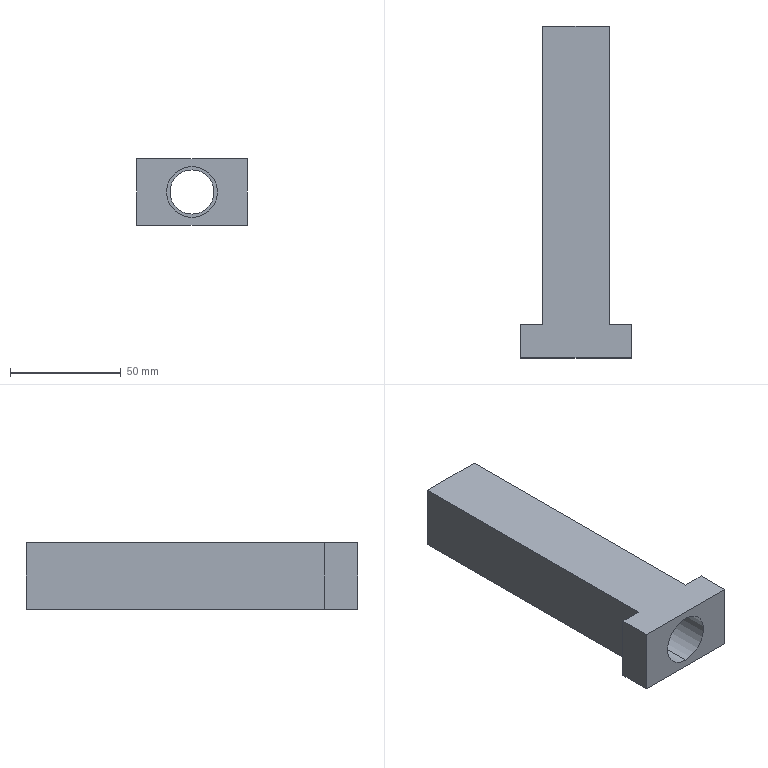Component | SolidWorks | Nut-1 | 1 solid | 15 faces | box 50 x 150 x 30 mm | volume 85731 mm3 | plane 11 | cylinder 4 | commonest cylinder face diameters 20 x2 23 x2
build123d program:
from build123d import *

# Parameters (mm, degrees)
SKETCH1_W           = 50
SKETCH1_H           = 30
BOSS_EXTRUDE1_DEPTH = 15
SKETCH2_W           = 30
SKETCH2_H           = 30
BOSS_EXTRUDE2_DEPTH = 135
CUT_EXTRUDE1_START  = -40
SKETCH3_R           = 11.5
CUT_EXTRUDE1_DEPTH  = 113.807
M20_TAPPED_HOLE1_D  = 20


with BuildPart() as part:
    # Sketch1 → Boss-Extrude1 (new body)
    with BuildSketch(Plane(origin=(0, 0, 0), x_dir=(1, 0, 0), z_dir=(0, 1, 0))):
        Rectangle(SKETCH1_W, SKETCH1_H)
    extrude(amount=BOSS_EXTRUDE1_DEPTH)

    # Sketch2 → Boss-Extrude2 (add)
    with BuildSketch(Plane(origin=(0, 15, 0), x_dir=(1, 0, 0), z_dir=(0, 1, 0))):
        Rectangle(SKETCH2_W, SKETCH2_H)
    extrude(amount=BOSS_EXTRUDE2_DEPTH)

    # Sketch3 → Cut-Extrude1 (cut, through all)
    with BuildSketch(Plane(origin=(0, 150, 0), x_dir=(1, 0, 0), z_dir=(0, 1, 0)).offset(CUT_EXTRUDE1_START)):
        with Locations(Location((0, 0, 0), (0, 0, 270))):
            Circle(SKETCH3_R)
    extrude(amount=-CUT_EXTRUDE1_DEPTH, mode=Mode.SUBTRACT)

    # M20 Tapped Hole1 (through all)
    with Locations(Plane(origin=(0, 150, 0), x_dir=(1, 0, 0), z_dir=(0, 1, 0))):
        with Locations((0, 0)):
            Hole(M20_TAPPED_HOLE1_D / 2)


solid = part.part

# Placed as in the assembly
solid = solid.moved(Location((-29.507, -119.411, 458), (0, 0, 0)))
STEP:
#1=COLOUR_RGB('',0.7922,0.8196,0.9333);
#2=FILL_AREA_STYLE_COLOUR('',#1);
#3=FILL_AREA_STYLE('',(#2));
#4=SURFACE_STYLE_FILL_AREA(#3);
#5=SURFACE_SIDE_STYLE('',(#4));
#6=SURFACE_STYLE_USAGE(.BOTH.,#5);
#7=PRESENTATION_STYLE_ASSIGNMENT((#6));
#8=CARTESIAN_POINT('',(-1.162,-0.3705,17.638));
#9=VERTEX_POINT('',#8);
#10=CARTESIAN_POINT('',(-1.162,-0.3705,18.425));
#11=VERTEX_POINT('',#10);
#12=CARTESIAN_POINT('',(-1.162,-0.3705,18.031));
#13=DIRECTION('',(0.,1.,0.));
#14=DIRECTION('',(0.,0.,1.));
#15=AXIS2_PLACEMENT_3D('',#12,#13,#14);
#16=CIRCLE('',#15,0.3937);
#17=EDGE_CURVE('',#9,#11,#16,.T.);
#18=ORIENTED_EDGE('',*,*,#17,.F.);
#19=CARTESIAN_POINT('',(-1.162,1.204,17.638));
#20=VERTEX_POINT('',#19);
#21=CARTESIAN_POINT('',(-1.162,1.204,17.638));
#22=DIRECTION('',(0.,1.,0.));
#23=VECTOR('',#22,39.37);
#24=LINE('',#21,#23);
#25=EDGE_CURVE('',#9,#20,#24,.T.);
#26=ORIENTED_EDGE('',*,*,#25,.T.);
#27=CARTESIAN_POINT('',(-1.162,1.204,18.425));
#28=VERTEX_POINT('',#27);
#29=CARTESIAN_POINT('',(-1.162,1.204,18.031));
#30=DIRECTION('',(0.,1.,0.));
#31=DIRECTION('',(0.,0.,1.));
#32=AXIS2_PLACEMENT_3D('',#29,#30,#31);
#33=CIRCLE('',#32,0.3937);
#34=EDGE_CURVE('',#20,#28,#33,.T.);
#35=ORIENTED_EDGE('',*,*,#34,.T.);
#36=CARTESIAN_POINT('',(-1.162,1.204,18.425));
#37=DIRECTION('',(0.,1.,0.));
#38=VECTOR('',#37,39.37);
#39=LINE('',#36,#38);
#40=EDGE_CURVE('',#11,#28,#39,.T.);
#41=ORIENTED_EDGE('',*,*,#40,.F.);
#42=EDGE_LOOP('',(#18,#26,#35,#41));
#43=FACE_OUTER_BOUND('',#42,.T.);
#44=CARTESIAN_POINT('',(-1.162,1.204,18.031));
#45=DIRECTION('',(0.,1.,0.));
#46=DIRECTION('',(0.,0.,1.));
#47=AXIS2_PLACEMENT_3D('',#44,#45,#46);
#48=CYLINDRICAL_SURFACE('',#47,0.3937);
#49=ADVANCED_FACE('',(#43),#48,.F.);
#50=CARTESIAN_POINT('',(-1.162,-4.701,17.579));
#51=VERTEX_POINT('',#50);
#52=CARTESIAN_POINT('',(-1.162,-4.701,18.484));
#53=VERTEX_POINT('',#52);
#54=CARTESIAN_POINT('',(-1.162,-4.701,18.031));
#55=DIRECTION('',(0.,1.,0.));
#56=DIRECTION('',(0.,0.,1.));
#57=AXIS2_PLACEMENT_3D('',#54,#55,#56);
#58=CIRCLE('',#57,0.4528);
#59=EDGE_CURVE('',#51,#53,#58,.T.);
#60=ORIENTED_EDGE('',*,*,#59,.F.);
#61=CARTESIAN_POINT('',(-1.162,-0.3705,17.579));
#62=VERTEX_POINT('',#61);
#63=CARTESIAN_POINT('',(-1.162,-4.701,17.579));
#64=DIRECTION('',(0.,1.,0.));
#65=VECTOR('',#64,39.37);
#66=LINE('',#63,#65);
#67=EDGE_CURVE('',#51,#62,#66,.T.);
#68=ORIENTED_EDGE('',*,*,#67,.T.);
#69=CARTESIAN_POINT('',(-1.162,-0.3705,18.484));
#70=VERTEX_POINT('',#69);
#71=CARTESIAN_POINT('',(-1.162,-0.3705,18.031));
#72=DIRECTION('',(0.,1.,0.));
#73=DIRECTION('',(0.,0.,1.));
#74=AXIS2_PLACEMENT_3D('',#71,#72,#73);
#75=CIRCLE('',#74,0.4528);
#76=EDGE_CURVE('',#62,#70,#75,.T.);
#77=ORIENTED_EDGE('',*,*,#76,.T.);
#78=CARTESIAN_POINT('',(-1.162,-4.701,18.484));
#79=DIRECTION('',(0.,1.,0.));
#80=VECTOR('',#79,39.37);
#81=LINE('',#78,#80);
#82=EDGE_CURVE('',#53,#70,#81,.T.);
#83=ORIENTED_EDGE('',*,*,#82,.F.);
#84=EDGE_LOOP('',(#60,#68,#77,#83));
#85=FACE_OUTER_BOUND('',#84,.T.);
#86=CARTESIAN_POINT('',(-1.162,-4.701,18.031));
#87=DIRECTION('',(0.,1.,0.));
#88=DIRECTION('',(0.,0.,1.));
#89=AXIS2_PLACEMENT_3D('',#86,#87,#88);
#90=CYLINDRICAL_SURFACE('',#89,0.4528);
#91=ADVANCED_FACE('',(#85),#90,.F.);
#92=CARTESIAN_POINT('',(-0.5711,-4.111,18.622));
#93=VERTEX_POINT('',#92);
#94=CARTESIAN_POINT('',(-0.5711,-4.111,17.441));
#95=VERTEX_POINT('',#94);
#96=CARTESIAN_POINT('',(-0.5711,-4.111,18.622));
#97=DIRECTION('',(0.,0.,-1.));
#98=VECTOR('',#97,39.37);
#99=LINE('',#96,#98);
#100=EDGE_CURVE('',#93,#95,#99,.T.);
#101=ORIENTED_EDGE('',*,*,#100,.F.);
#102=CARTESIAN_POINT('',(-0.1774,-4.111,18.622));
#103=VERTEX_POINT('',#102);
#104=CARTESIAN_POINT('',(-2.146,-4.111,18.622));
#105=DIRECTION('',(1.,0.,0.));
#106=VECTOR('',#105,39.37);
#107=LINE('',#104,#106);
#108=EDGE_CURVE('',#93,#103,#107,.T.);
#109=ORIENTED_EDGE('',*,*,#108,.T.);
#110=CARTESIAN_POINT('',(-0.1774,-4.111,17.441));
#111=VERTEX_POINT('',#110);
#112=CARTESIAN_POINT('',(-0.1774,-4.111,17.441));
#113=DIRECTION('',(-0.,0.,-1.));
#114=VECTOR('',#113,39.37);
#115=LINE('',#112,#114);
#116=EDGE_CURVE('',#103,#111,#115,.T.);
#117=ORIENTED_EDGE('',*,*,#116,.T.);
#118=CARTESIAN_POINT('',(-2.146,-4.111,17.441));
#119=DIRECTION('',(-1.,0.,0.));
#120=VECTOR('',#119,39.37);
#121=LINE('',#118,#120);
#122=EDGE_CURVE('',#111,#95,#121,.T.);
#123=ORIENTED_EDGE('',*,*,#122,.T.);
#124=EDGE_LOOP('',(#101,#109,#117,#123));
#125=FACE_OUTER_BOUND('',#124,.T.);
#126=CARTESIAN_POINT('',(-1.162,-4.111,18.031));
#127=DIRECTION('',(0.,1.,0.));
#128=DIRECTION('',(0.,0.,1.));
#129=AXIS2_PLACEMENT_3D('',#126,#127,#128);
#130=PLANE('',#129);
#131=ADVANCED_FACE('',(#125),#130,.T.);
#132=CARTESIAN_POINT('',(-0.1774,-4.701,18.622));
#133=VERTEX_POINT('',#132);
#134=CARTESIAN_POINT('',(-0.1774,-4.701,17.441));
#135=VERTEX_POINT('',#134);
#136=CARTESIAN_POINT('',(-0.1774,-4.701,17.441));
#137=DIRECTION('',(-0.,0.,-1.));
#138=VECTOR('',#137,39.37);
#139=LINE('',#136,#138);
#140=EDGE_CURVE('',#133,#135,#139,.T.);
#141=ORIENTED_EDGE('',*,*,#140,.T.);
#142=CARTESIAN_POINT('',(-0.1774,-4.111,17.441));
#143=DIRECTION('',(0.,-1.,0.));
#144=VECTOR('',#143,39.37);
#145=LINE('',#142,#144);
#146=EDGE_CURVE('',#111,#135,#145,.T.);
#147=ORIENTED_EDGE('',*,*,#146,.F.);
#148=ORIENTED_EDGE('',*,*,#116,.F.);
#149=CARTESIAN_POINT('',(-0.1774,-4.111,18.622));
#150=DIRECTION('',(0.,-1.,0.));
#151=VECTOR('',#150,39.37);
#152=LINE('',#149,#151);
#153=EDGE_CURVE('',#103,#133,#152,.T.);
#154=ORIENTED_EDGE('',*,*,#153,.T.);
#155=EDGE_LOOP('',(#141,#147,#148,#154));
#156=FACE_OUTER_BOUND('',#155,.T.);
#157=CARTESIAN_POINT('',(-0.1774,-4.111,17.441));
#158=DIRECTION('',(-1.,0.,0.));
#159=DIRECTION('',(0.,0.,1.));
#160=AXIS2_PLACEMENT_3D('',#157,#158,#159);
#161=PLANE('',#160);
#162=ADVANCED_FACE('',(#156),#161,.F.);
#163=CARTESIAN_POINT('',(-2.146,-4.701,17.441));
#164=VERTEX_POINT('',#163);
#165=CARTESIAN_POINT('',(-2.146,-4.701,17.441));
#166=DIRECTION('',(-1.,0.,0.));
#167=VECTOR('',#166,39.37);
#168=LINE('',#165,#167);
#169=EDGE_CURVE('',#135,#164,#168,.T.);
#170=ORIENTED_EDGE('',*,*,#169,.T.);
#171=CARTESIAN_POINT('',(-2.146,-4.111,17.441));
#172=VERTEX_POINT('',#171);
#173=CARTESIAN_POINT('',(-2.146,-4.111,17.441));
#174=DIRECTION('',(0.,-1.,0.));
#175=VECTOR('',#174,39.37);
#176=LINE('',#173,#175);
#177=EDGE_CURVE('',#172,#164,#176,.T.);
#178=ORIENTED_EDGE('',*,*,#177,.F.);
#179=CARTESIAN_POINT('',(-1.752,-4.111,17.441));
#180=VERTEX_POINT('',#179);
#181=CARTESIAN_POINT('',(-2.146,-4.111,17.441));
#182=DIRECTION('',(-1.,0.,0.));
#183=VECTOR('',#182,39.37);
#184=LINE('',#181,#183);
#185=EDGE_CURVE('',#180,#172,#184,.T.);
#186=ORIENTED_EDGE('',*,*,#185,.F.);
#187=CARTESIAN_POINT('',(-1.752,1.204,17.441));
#188=VERTEX_POINT('',#187);
#189=CARTESIAN_POINT('',(-1.752,1.204,17.441));
#190=DIRECTION('',(0.,-1.,0.));
#191=VECTOR('',#190,39.37);
#192=LINE('',#189,#191);
#193=EDGE_CURVE('',#188,#180,#192,.T.);
#194=ORIENTED_EDGE('',*,*,#193,.F.);
#195=CARTESIAN_POINT('',(-0.5711,1.204,17.441));
#196=VERTEX_POINT('',#195);
#197=CARTESIAN_POINT('',(-1.752,1.204,17.441));
#198=DIRECTION('',(-1.,0.,0.));
#199=VECTOR('',#198,39.37);
#200=LINE('',#197,#199);
#201=EDGE_CURVE('',#196,#188,#200,.T.);
#202=ORIENTED_EDGE('',*,*,#201,.F.);
#203=CARTESIAN_POINT('',(-0.5711,1.204,17.441));
#204=DIRECTION('',(0.,-1.,0.));
#205=VECTOR('',#204,39.37);
#206=LINE('',#203,#205);
#207=EDGE_CURVE('',#196,#95,#206,.T.);
#208=ORIENTED_EDGE('',*,*,#207,.T.);
#209=ORIENTED_EDGE('',*,*,#122,.F.);
#210=ORIENTED_EDGE('',*,*,#146,.T.);
#211=EDGE_LOOP('',(#170,#178,#186,#194,#202,#208,#209,#210));
#212=FACE_OUTER_BOUND('',#211,.T.);
#213=CARTESIAN_POINT('',(-2.146,-4.111,17.441));
#214=DIRECTION('',(0.,0.,1.));
#215=DIRECTION('',(1.,0.,0.));
#216=AXIS2_PLACEMENT_3D('',#213,#214,#215);
#217=PLANE('',#216);
#218=ADVANCED_FACE('',(#212),#217,.F.);
#219=CARTESIAN_POINT('',(-2.146,-4.701,18.622));
#220=VERTEX_POINT('',#219);
#221=CARTESIAN_POINT('',(-2.146,-4.701,17.441));
#222=DIRECTION('',(0.,0.,1.));
#223=VECTOR('',#222,39.37);
#224=LINE('',#221,#223);
#225=EDGE_CURVE('',#164,#220,#224,.T.);
#226=ORIENTED_EDGE('',*,*,#225,.T.);
#227=CARTESIAN_POINT('',(-2.146,-4.111,18.622));
#228=VERTEX_POINT('',#227);
#229=CARTESIAN_POINT('',(-2.146,-4.111,18.622));
#230=DIRECTION('',(0.,-1.,0.));
#231=VECTOR('',#230,39.37);
#232=LINE('',#229,#231);
#233=EDGE_CURVE('',#228,#220,#232,.T.);
#234=ORIENTED_EDGE('',*,*,#233,.F.);
#235=CARTESIAN_POINT('',(-2.146,-4.111,17.441));
#236=DIRECTION('',(0.,0.,1.));
#237=VECTOR('',#236,39.37);
#238=LINE('',#235,#237);
#239=EDGE_CURVE('',#172,#228,#238,.T.);
#240=ORIENTED_EDGE('',*,*,#239,.F.);
#241=ORIENTED_EDGE('',*,*,#177,.T.);
#242=EDGE_LOOP('',(#226,#234,#240,#241));
#243=FACE_OUTER_BOUND('',#242,.T.);
#244=CARTESIAN_POINT('',(-2.146,-4.111,17.441));
#245=DIRECTION('',(1.,0.,-0.));
#246=DIRECTION('',(-0.,0.,-1.));
#247=AXIS2_PLACEMENT_3D('',#244,#245,#246);
#248=PLANE('',#247);
#249=ADVANCED_FACE('',(#243),#248,.F.);
#250=CARTESIAN_POINT('',(-2.146,-4.701,18.622));
#251=DIRECTION('',(1.,0.,0.));
#252=VECTOR('',#251,39.37);
#253=LINE('',#250,#252);
#254=EDGE_CURVE('',#220,#133,#253,.T.);
#255=ORIENTED_EDGE('',*,*,#254,.T.);
#256=ORIENTED_EDGE('',*,*,#153,.F.);
#257=ORIENTED_EDGE('',*,*,#108,.F.);
#258=CARTESIAN_POINT('',(-0.5711,1.204,18.622));
#259=VERTEX_POINT('',#258);
#260=CARTESIAN_POINT('',(-0.5711,1.204,18.622));
#261=DIRECTION('',(0.,-1.,0.));
#262=VECTOR('',#261,39.37);
#263=LINE('',#260,#262);
#264=EDGE_CURVE('',#259,#93,#263,.T.);
#265=ORIENTED_EDGE('',*,*,#264,.F.);
#266=CARTESIAN_POINT('',(-1.752,1.204,18.622));
#267=VERTEX_POINT('',#266);
#268=CARTESIAN_POINT('',(-1.752,1.204,18.622));
#269=DIRECTION('',(1.,0.,0.));
#270=VECTOR('',#269,39.37);
#271=LINE('',#268,#270);
#272=EDGE_CURVE('',#267,#259,#271,.T.);
#273=ORIENTED_EDGE('',*,*,#272,.F.);
#274=CARTESIAN_POINT('',(-1.752,-4.111,18.622));
#275=VERTEX_POINT('',#274);
#276=CARTESIAN_POINT('',(-1.752,1.204,18.622));
#277=DIRECTION('',(0.,-1.,0.));
#278=VECTOR('',#277,39.37);
#279=LINE('',#276,#278);
#280=EDGE_CURVE('',#267,#275,#279,.T.);
#281=ORIENTED_EDGE('',*,*,#280,.T.);
#282=CARTESIAN_POINT('',(-2.146,-4.111,18.622));
#283=DIRECTION('',(1.,0.,0.));
#284=VECTOR('',#283,39.37);
#285=LINE('',#282,#284);
#286=EDGE_CURVE('',#228,#275,#285,.T.);
#287=ORIENTED_EDGE('',*,*,#286,.F.);
#288=ORIENTED_EDGE('',*,*,#233,.T.);
#289=EDGE_LOOP('',(#255,#256,#257,#265,#273,#281,#287,#288));
#290=FACE_OUTER_BOUND('',#289,.T.);
#291=CARTESIAN_POINT('',(-2.146,-4.111,18.622));
#292=DIRECTION('',(0.,0.,-1.));
#293=DIRECTION('',(-1.,0.,0.));
#294=AXIS2_PLACEMENT_3D('',#291,#292,#293);
#295=PLANE('',#294);
#296=ADVANCED_FACE('',(#290),#295,.F.);
#297=CARTESIAN_POINT('',(-1.752,-4.111,18.622));
#298=DIRECTION('',(0.,0.,1.));
#299=VECTOR('',#298,39.37);
#300=LINE('',#297,#299);
#301=EDGE_CURVE('',#180,#275,#300,.T.);
#302=ORIENTED_EDGE('',*,*,#301,.F.);
#303=ORIENTED_EDGE('',*,*,#185,.T.);
#304=ORIENTED_EDGE('',*,*,#239,.T.);
#305=ORIENTED_EDGE('',*,*,#286,.T.);
#306=EDGE_LOOP('',(#302,#303,#304,#305));
#307=FACE_OUTER_BOUND('',#306,.T.);
#308=CARTESIAN_POINT('',(-1.162,-4.111,18.031));
#309=DIRECTION('',(0.,1.,0.));
#310=DIRECTION('',(0.,0.,1.));
#311=AXIS2_PLACEMENT_3D('',#308,#309,#310);
#312=PLANE('',#311);
#313=ADVANCED_FACE('',(#307),#312,.T.);
#314=CARTESIAN_POINT('',(-1.162,-4.701,18.031));
#315=DIRECTION('',(0.,1.,0.));
#316=DIRECTION('',(0.,0.,1.));
#317=AXIS2_PLACEMENT_3D('',#314,#315,#316);
#318=CIRCLE('',#317,0.4528);
#319=EDGE_CURVE('',#53,#51,#318,.T.);
#320=ORIENTED_EDGE('',*,*,#319,.T.);
#321=ORIENTED_EDGE('',*,*,#59,.T.);
#322=EDGE_LOOP('',(#320,#321));
#323=FACE_BOUND('',#322,.T.);
#324=ORIENTED_EDGE('',*,*,#140,.F.);
#325=ORIENTED_EDGE('',*,*,#254,.F.);
#326=ORIENTED_EDGE('',*,*,#225,.F.);
#327=ORIENTED_EDGE('',*,*,#169,.F.);
#328=EDGE_LOOP('',(#324,#325,#326,#327));
#329=FACE_OUTER_BOUND('',#328,.T.);
#330=CARTESIAN_POINT('',(-1.162,-4.701,18.031));
#331=DIRECTION('',(0.,1.,0.));
#332=DIRECTION('',(0.,0.,1.));
#333=AXIS2_PLACEMENT_3D('',#330,#331,#332);
#334=PLANE('',#333);
#335=ADVANCED_FACE('',(#323,#329),#334,.F.);
#336=ORIENTED_EDGE('',*,*,#100,.T.);
#337=ORIENTED_EDGE('',*,*,#207,.F.);
#338=CARTESIAN_POINT('',(-0.5711,1.204,18.622));
#339=DIRECTION('',(0.,0.,-1.));
#340=VECTOR('',#339,39.37);
#341=LINE('',#338,#340);
#342=EDGE_CURVE('',#259,#196,#341,.T.);
#343=ORIENTED_EDGE('',*,*,#342,.F.);
#344=ORIENTED_EDGE('',*,*,#264,.T.);
#345=EDGE_LOOP('',(#336,#337,#343,#344));
#346=FACE_OUTER_BOUND('',#345,.T.);
#347=CARTESIAN_POINT('',(-0.5711,1.204,18.622));
#348=DIRECTION('',(-1.,0.,0.));
#349=DIRECTION('',(0.,0.,1.));
#350=AXIS2_PLACEMENT_3D('',#347,#348,#349);
#351=PLANE('',#350);
#352=ADVANCED_FACE('',(#346),#351,.F.);
#353=ORIENTED_EDGE('',*,*,#301,.T.);
#354=ORIENTED_EDGE('',*,*,#280,.F.);
#355=CARTESIAN_POINT('',(-1.752,1.204,18.622));
#356=DIRECTION('',(0.,0.,1.));
#357=VECTOR('',#356,39.37);
#358=LINE('',#355,#357);
#359=EDGE_CURVE('',#188,#267,#358,.T.);
#360=ORIENTED_EDGE('',*,*,#359,.F.);
#361=ORIENTED_EDGE('',*,*,#193,.T.);
#362=EDGE_LOOP('',(#353,#354,#360,#361));
#363=FACE_OUTER_BOUND('',#362,.T.);
#364=CARTESIAN_POINT('',(-1.752,1.204,18.622));
#365=DIRECTION('',(1.,0.,0.));
#366=DIRECTION('',(0.,0.,-1.));
#367=AXIS2_PLACEMENT_3D('',#364,#365,#366);
#368=PLANE('',#367);
#369=ADVANCED_FACE('',(#363),#368,.F.);
#370=CARTESIAN_POINT('',(-1.162,1.204,18.031));
#371=DIRECTION('',(0.,1.,0.));
#372=DIRECTION('',(0.,0.,1.));
#373=AXIS2_PLACEMENT_3D('',#370,#371,#372);
#374=CIRCLE('',#373,0.3937);
#375=EDGE_CURVE('',#28,#20,#374,.T.);
#376=ORIENTED_EDGE('',*,*,#375,.F.);
#377=ORIENTED_EDGE('',*,*,#34,.F.);
#378=EDGE_LOOP('',(#376,#377));
#379=FACE_BOUND('',#378,.T.);
#380=ORIENTED_EDGE('',*,*,#342,.T.);
#381=ORIENTED_EDGE('',*,*,#201,.T.);
#382=ORIENTED_EDGE('',*,*,#359,.T.);
#383=ORIENTED_EDGE('',*,*,#272,.T.);
#384=EDGE_LOOP('',(#380,#381,#382,#383));
#385=FACE_OUTER_BOUND('',#384,.T.);
#386=CARTESIAN_POINT('',(-1.162,1.204,18.031));
#387=DIRECTION('',(0.,-1.,0.));
#388=DIRECTION('',(0.,0.,-1.));
#389=AXIS2_PLACEMENT_3D('',#386,#387,#388);
#390=PLANE('',#389);
#391=ADVANCED_FACE('',(#379,#385),#390,.F.);
#392=ORIENTED_EDGE('',*,*,#67,.F.);
#393=ORIENTED_EDGE('',*,*,#319,.F.);
#394=ORIENTED_EDGE('',*,*,#82,.T.);
#395=CARTESIAN_POINT('',(-1.162,-0.3705,18.031));
#396=DIRECTION('',(0.,1.,0.));
#397=DIRECTION('',(0.,0.,1.));
#398=AXIS2_PLACEMENT_3D('',#395,#396,#397);
#399=CIRCLE('',#398,0.4528);
#400=EDGE_CURVE('',#70,#62,#399,.T.);
#401=ORIENTED_EDGE('',*,*,#400,.T.);
#402=EDGE_LOOP('',(#392,#393,#394,#401));
#403=FACE_OUTER_BOUND('',#402,.T.);
#404=CARTESIAN_POINT('',(-1.162,-4.701,18.031));
#405=DIRECTION('',(0.,1.,0.));
#406=DIRECTION('',(0.,0.,1.));
#407=AXIS2_PLACEMENT_3D('',#404,#405,#406);
#408=CYLINDRICAL_SURFACE('',#407,0.4528);
#409=ADVANCED_FACE('',(#403),#408,.F.);
#410=CARTESIAN_POINT('',(-1.162,-0.3705,18.031));
#411=DIRECTION('',(0.,1.,0.));
#412=DIRECTION('',(0.,0.,1.));
#413=AXIS2_PLACEMENT_3D('',#410,#411,#412);
#414=CIRCLE('',#413,0.3937);
#415=EDGE_CURVE('',#11,#9,#414,.T.);
#416=ORIENTED_EDGE('',*,*,#415,.T.);
#417=ORIENTED_EDGE('',*,*,#17,.T.);
#418=EDGE_LOOP('',(#416,#417));
#419=FACE_BOUND('',#418,.T.);
#420=ORIENTED_EDGE('',*,*,#400,.F.);
#421=ORIENTED_EDGE('',*,*,#76,.F.);
#422=EDGE_LOOP('',(#420,#421));
#423=FACE_OUTER_BOUND('',#422,.T.);
#424=CARTESIAN_POINT('',(-1.162,-0.3705,18.031));
#425=DIRECTION('',(0.,1.,0.));
#426=DIRECTION('',(0.,0.,1.));
#427=AXIS2_PLACEMENT_3D('',#424,#425,#426);
#428=PLANE('',#427);
#429=ADVANCED_FACE('',(#419,#423),#428,.F.);
#430=ORIENTED_EDGE('',*,*,#25,.F.);
#431=ORIENTED_EDGE('',*,*,#415,.F.);
#432=ORIENTED_EDGE('',*,*,#40,.T.);
#433=ORIENTED_EDGE('',*,*,#375,.T.);
#434=EDGE_LOOP('',(#430,#431,#432,#433));
#435=FACE_OUTER_BOUND('',#434,.T.);
#436=CARTESIAN_POINT('',(-1.162,1.204,18.031));
#437=DIRECTION('',(0.,1.,0.));
#438=DIRECTION('',(0.,0.,1.));
#439=AXIS2_PLACEMENT_3D('',#436,#437,#438);
#440=CYLINDRICAL_SURFACE('',#439,0.3937);
#441=ADVANCED_FACE('',(#435),#440,.F.);
#442=CLOSED_SHELL('',(#49,#91,#131,#162,#218,#249,#296,#313,#335,#352,#369,#391,#409,#429,#441));
#443=MANIFOLD_SOLID_BREP('',#442);
#444=STYLED_ITEM('',(#7),#443);
#445=(LENGTH_UNIT()NAMED_UNIT(*)SI_UNIT($,.METRE.));
#446=LENGTH_MEASURE_WITH_UNIT(LENGTH_MEASURE(0.0254),#445);
#447=DIMENSIONAL_EXPONENTS(1.,0.,0.,0.,0.,0.,0.);
#448=(CONVERSION_BASED_UNIT('',#446)LENGTH_UNIT()NAMED_UNIT(#447));
#449=UNCERTAINTY_MEASURE_WITH_UNIT(LENGTH_MEASURE(0.00001),#448,'','');
#450=(NAMED_UNIT(*)PLANE_ANGLE_UNIT()SI_UNIT($,.RADIAN.));
#451=(NAMED_UNIT(*)SI_UNIT($,.STERADIAN.)SOLID_ANGLE_UNIT());
#452=(GEOMETRIC_REPRESENTATION_CONTEXT(3)GLOBAL_UNCERTAINTY_ASSIGNED_CONTEXT((#449))GLOBAL_UNIT_ASSIGNED_CONTEXT((#448,#450,#451))REPRESENTATION_CONTEXT('',''));
#453=MECHANICAL_DESIGN_GEOMETRIC_PRESENTATION_REPRESENTATION('',(#444),#452);
#454=CARTESIAN_POINT('',(0.,0.,0.));
#455=DIRECTION('',(0.,0.,1.));
#456=DIRECTION('',(1.,0.,0.));
#457=AXIS2_PLACEMENT_3D('',#454,#455,#456);
#458=(LENGTH_UNIT()NAMED_UNIT(*)SI_UNIT($,.METRE.));
#459=LENGTH_MEASURE_WITH_UNIT(LENGTH_MEASURE(0.0254),#458);
#460=DIMENSIONAL_EXPONENTS(1.,0.,0.,0.,0.,0.,0.);
#461=(CONVERSION_BASED_UNIT('',#459)LENGTH_UNIT()NAMED_UNIT(#460));
#462=UNCERTAINTY_MEASURE_WITH_UNIT(LENGTH_MEASURE(0.00001),#461,'','');
#463=(NAMED_UNIT(*)PLANE_ANGLE_UNIT()SI_UNIT($,.RADIAN.));
#464=(NAMED_UNIT(*)SI_UNIT($,.STERADIAN.)SOLID_ANGLE_UNIT());
#465=(GEOMETRIC_REPRESENTATION_CONTEXT(3)GLOBAL_UNCERTAINTY_ASSIGNED_CONTEXT((#462))GLOBAL_UNIT_ASSIGNED_CONTEXT((#461,#463,#464))REPRESENTATION_CONTEXT('',''));
#466=ADVANCED_BREP_SHAPE_REPRESENTATION('',(#443,#457),#465);
#467=PRESENTATION_LAYER_ASSIGNMENT('','',(#444));